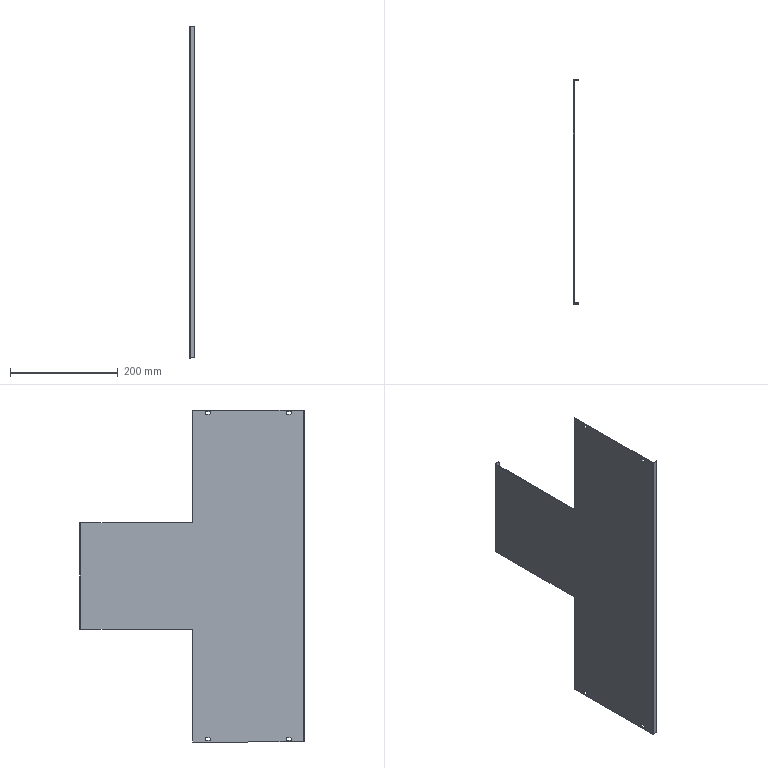Component | SolidWorks | PG50-06(BottomPlateWeldingDrawing)-1_BottomPlateWeldment1(PG50-06-101-1 | 1 solid | 42 faces | volume 262048 mm3 | plane 30 | cylinder 12 | commonest cylinder face diameters 5 x8 3.3 x2 0.3 x2 | material AISI 1045 Steel, cold drawn